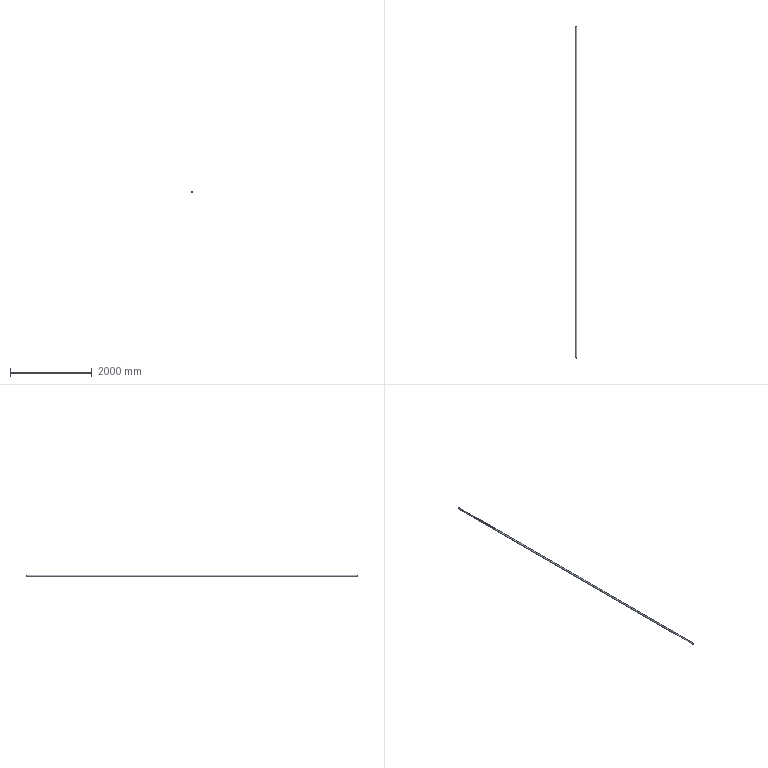Component | NX | 43_3_2 | 1 solid | 4 faces | volume 2716457 mm3 | cylinder 2 | plane 2 | commonest cylinder face diameters 34 x1 27 x1